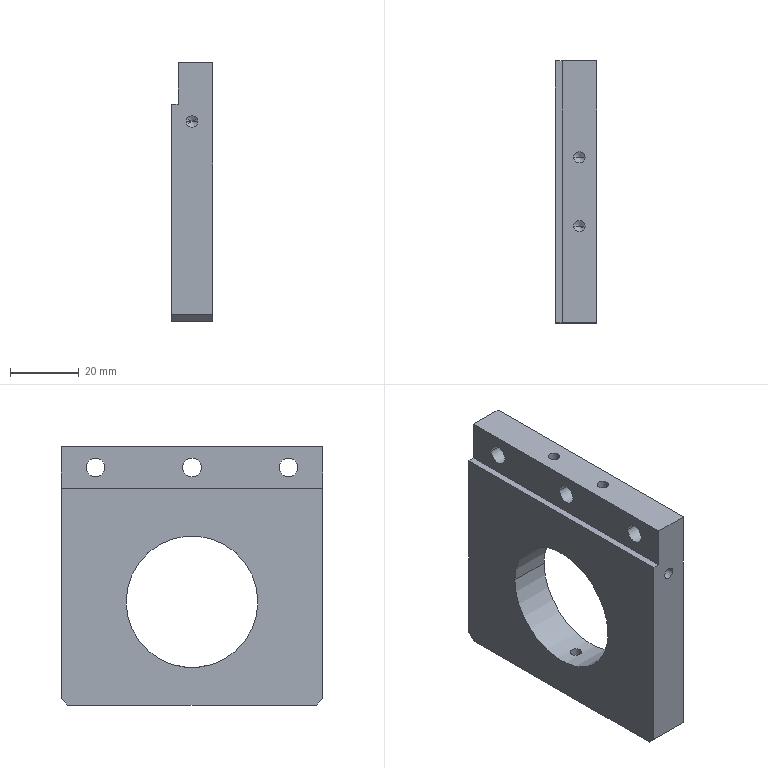Component | SolidWorks | UpperServoSeat-2-1 | 1 solid | 45 faces | box 12 x 76 x 75 mm | volume 50742 mm3 | cylinder 24 | plane 13 | cone 8 | commonest cylinder face diameters 3.3 x10 10 x6 5.5 x6 38.2 x2
build123d program:
from build123d import *

# Parameters (mm, degrees)
SKETCH1_W                                            = 76
SKETCH1_H                                            = 75
BOSS_EXTRUDE1_DEPTH                                  = 12
SKETCH2_W                                            = 76
SKETCH2_H                                            = 12
CUT_EXTRUDE1_DEPTH                                   = 2
SKETCH7_R                                            = 19.1
CUT_EXTRUDE4_DEPTH                                   = 15
CYLINDRICAL_COUNTERSUNK_HOLE_FOR_M5_SOCK_D           = 5.5
CYLINDRICAL_COUNTERSUNK_HOLE_FOR_M5_SOCK_CBORE_D     = 10
CYLINDRICAL_COUNTERSUNK_HOLE_FOR_M5_SOCK_CBORE_DEPTH = 5
CHAMFER1_SIZE                                        = 2
M4_TAPPED_HOLE2_D                                    = 3.3
M4_TAPPED_HOLE2_DEPTH                                = 11.5
M4_TAPPED_HOLE2_TIP                                  = 0.9914
M4_TAPPED_HOLE3_D                                    = 3.3
M4_TAPPED_HOLE3_DEPTH                                = 11.5
M4_TAPPED_HOLE3_TIP                                  = 0.9914
M4_TAPPED_HOLE4_D                                    = 3.3
M4_TAPPED_HOLE4_DEPTH                                = 11.5
M4_TAPPED_HOLE4_TIP                                  = 0.9914
M4_TAPPED_HOLE5_D                                    = 3.3
M4_TAPPED_HOLE5_DEPTH                                = 11.5
M4_TAPPED_HOLE5_TIP                                  = 0.9914


with BuildPart() as part:
    # Sketch1 → Boss-Extrude1 (new body)
    with BuildSketch(Plane.XY):
        with Locations((38, 37.5)):
            Rectangle(SKETCH1_W, SKETCH1_H)
    extrude(amount=BOSS_EXTRUDE1_DEPTH)

    # Sketch2 → Cut-Extrude1 (cut)
    with BuildSketch(Plane.XY.offset(12)):
        with Locations((38, 6)):
            Rectangle(SKETCH2_W, SKETCH2_H)
    extrude(amount=-CUT_EXTRUDE1_DEPTH, mode=Mode.SUBTRACT)

    # Sketch7 → Cut-Extrude4 (cut)
    with BuildSketch(Plane(origin=(0, 0, 0), x_dir=(-1, 0, 0), z_dir=(0, 0, -1))):
        with Locations((-38, 45)):
            Circle(SKETCH7_R)
    extrude(amount=-CUT_EXTRUDE4_DEPTH, mode=Mode.SUBTRACT)

    # Cylindrical Countersunk Hole for M5 Sock (through all)
    with Locations(Plane(origin=(0, 0, 0), x_dir=(-1, 0, 0), z_dir=(0, 0, -1))):
        with Locations((-66, 6), (-38, 6), (-10, 6)):
            CounterBoreHole(CYLINDRICAL_COUNTERSUNK_HOLE_FOR_M5_SOCK_D / 2, CYLINDRICAL_COUNTERSUNK_HOLE_FOR_M5_SOCK_CBORE_D / 2, CYLINDRICAL_COUNTERSUNK_HOLE_FOR_M5_SOCK_CBORE_DEPTH)

    # Chamfer1
    chamfer1_edges = [part.edges().sort_by_distance(p)[0] for p in [
        (0, 75, 6),
        (76, 75, 6),
    ]]
    chamfer(chamfer1_edges, length=CHAMFER1_SIZE)

    # M4 Tapped Hole2
    with Locations(Plane.ZY):
        with Locations((6, 17)):
            Hole(M4_TAPPED_HOLE2_D / 2, depth=M4_TAPPED_HOLE2_DEPTH)
            with Locations((0, 0, -(M4_TAPPED_HOLE2_DEPTH + M4_TAPPED_HOLE2_TIP / 2))):  # 118° drill point
                Cone(0, M4_TAPPED_HOLE2_D / 2, M4_TAPPED_HOLE2_TIP, mode=Mode.SUBTRACT)

    # M4 Tapped Hole3
    with Locations(Plane(origin=(0, 75, 0), x_dir=(1, 0, 0), z_dir=(0, 1, 0))):
        with Locations((38, -6)):
            Hole(M4_TAPPED_HOLE3_D / 2, depth=M4_TAPPED_HOLE3_DEPTH)
            with Locations((0, 0, -(M4_TAPPED_HOLE3_DEPTH + M4_TAPPED_HOLE3_TIP / 2))):  # 118° drill point
                Cone(0, M4_TAPPED_HOLE3_D / 2, M4_TAPPED_HOLE3_TIP, mode=Mode.SUBTRACT)

    # M4 Tapped Hole4
    with Locations(Plane(origin=(76, 0, 0), x_dir=(0, 0, -1), z_dir=(1, 0, 0))):
        with Locations((-6, 17)):
            Hole(M4_TAPPED_HOLE4_D / 2, depth=M4_TAPPED_HOLE4_DEPTH)
            with Locations((0, 0, -(M4_TAPPED_HOLE4_DEPTH + M4_TAPPED_HOLE4_TIP / 2))):  # 118° drill point
                Cone(0, M4_TAPPED_HOLE4_D / 2, M4_TAPPED_HOLE4_TIP, mode=Mode.SUBTRACT)

    # M4 Tapped Hole5
    with Locations(Plane(origin=(0, 0, 0), x_dir=(-1, 0, 0), z_dir=(0, -1, 0))):
        with Locations((-48, -5), (-28, -5)):
            Hole(M4_TAPPED_HOLE5_D / 2, depth=M4_TAPPED_HOLE5_DEPTH)
            with Locations((0, 0, -(M4_TAPPED_HOLE5_DEPTH + M4_TAPPED_HOLE5_TIP / 2))):  # 118° drill point
                Cone(0, M4_TAPPED_HOLE5_D / 2, M4_TAPPED_HOLE5_TIP, mode=Mode.SUBTRACT)


solid = part.part

# Placed as in the assembly
solid = solid.moved(Location((104.478, -18.055, 48.551), (-90, -90, 0)))